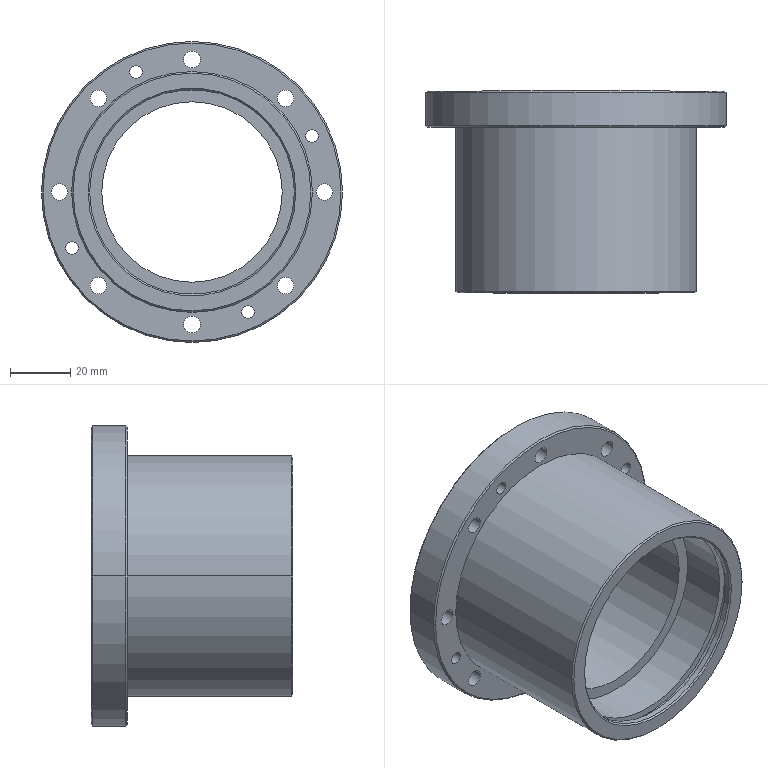Component | SolidWorks | BearingHousingAssembly-1_BearingHolder-1 | 1 solid | 85 faces | box 100 x 67 x 100 mm | volume 140911 mm3 | cylinder 58 | plane 17 | cone 10 | commonest cylinder face diameters 10 x16 5.5 x16 4.2 x8 68 x8 72.5 x4 80 x2 100 x2 60 x2 | material Plain Carbon Steel
build123d program:
from build123d import *

# Parameters (mm, degrees)
SKETCH1_R                                          = 50
BOSS_EXTRUDE1_DEPTH                                = 12
SKETCH2_R                                          = 40
BOSS_EXTRUDE2_DEPTH                                = 55
HOLE_SIZE_ACCORDING_TO_TYPE_OF_HEXAGON_D           = 5.5
HOLE_SIZE_ACCORDING_TO_TYPE_OF_HEXAGON_CBORE_D     = 10
HOLE_SIZE_ACCORDING_TO_TYPE_OF_HEXAGON_CBORE_DEPTH = 5.7
CIRPATTERN1_COUNT                                  = 8
SKETCH6_R                                          = 30
CUT_EXTRUDE1_DEPTH                                 = 98.411
SKETCH7_R                                          = 34
CUT_EXTRUDE2_DEPTH                                 = 20
CUT_EXTRUDE3_START                                 = -20
SKETCH8_R                                          = 34
CUT_EXTRUDE3_DEPTH                                 = 20
CHAMFER1_SIZE                                      = 0.5
SKETCH9_W                                          = 2.6
SKETCH9_H                                          = 2.25
M5_TAPPED_HOLE1_D                                  = 4.2
CIRPATTERN2_COUNT                                  = 4


with BuildPart() as part:
    # Sketch1 → Boss-Extrude1 (new body)
    with BuildSketch(Plane.XY):
        Circle(SKETCH1_R)
    extrude(amount=BOSS_EXTRUDE1_DEPTH)

    # Sketch2 → Boss-Extrude2 (add)
    with BuildSketch(Plane.XY.offset(12)):
        Circle(SKETCH2_R)
    extrude(amount=BOSS_EXTRUDE2_DEPTH)

    # Hole Size _according to_ type of Hexagon (through all)
    with Locations(Plane(origin=(0, 0, 0), x_dir=(-1, 0, 0), z_dir=(0, 0, -1))):
        with Locations((0, 44)):
            hole_size_according_to_type_of_hexagon = CounterBoreHole(HOLE_SIZE_ACCORDING_TO_TYPE_OF_HEXAGON_D / 2, HOLE_SIZE_ACCORDING_TO_TYPE_OF_HEXAGON_CBORE_D / 2, HOLE_SIZE_ACCORDING_TO_TYPE_OF_HEXAGON_CBORE_DEPTH)

    # CirPattern1: Hole Size _according to_ type of Hexagon ×8 about axis
    cirpattern1_axis = Axis((0, 0, 0), (0, 0, 1))
    for i in range(1, CIRPATTERN1_COUNT):
        add(hole_size_according_to_type_of_hexagon.rotate(cirpattern1_axis, i * 360 / CIRPATTERN1_COUNT), mode=Mode.SUBTRACT)

    # Sketch6 → Cut-Extrude1 (cut, through all)
    with BuildSketch(Plane.XY.offset(67)):
        Circle(SKETCH6_R)
    extrude(amount=-CUT_EXTRUDE1_DEPTH, mode=Mode.SUBTRACT)

    # Sketch7 → Cut-Extrude2 (cut)
    with BuildSketch(Plane.XY.offset(67)):
        Circle(SKETCH7_R)
    extrude(amount=-CUT_EXTRUDE2_DEPTH, mode=Mode.SUBTRACT)

    # Sketch8 → Cut-Extrude3 (cut)
    with BuildSketch(Plane(origin=(0, 0, 0), x_dir=(-1, 0, 0), z_dir=(0, 0, -1)).offset(CUT_EXTRUDE3_START)):
        with Locations(Location((0, 0, 0), (0, 0, 180))):
            Circle(SKETCH8_R)
    extrude(amount=CUT_EXTRUDE3_DEPTH, mode=Mode.SUBTRACT)

    # Chamfer1
    chamfer1_edges = [part.edges().sort_by_distance(p)[0] for p in [
        (-50, 0, 0),
        (-50, 0, 12),
        (-40, 0, 67),
        (-34, 0, 67),
        (-34, 0, 0),
    ]]
    chamfer(chamfer1_edges, length=CHAMFER1_SIZE)

    # Sketch9 → Cut-Revolve1 (revolve, cut)
    with BuildSketch(Plane(origin=(0, 0, 0), x_dir=(0, 0, -1), z_dir=(1, 0, 0)), mode=Mode.PRIVATE) as cut_revolve1_sk:
        with Locations((-63.3, 35.125)):
            Rectangle(SKETCH9_W, SKETCH9_H)
        with Locations((-3.7, 35.125)):
            Rectangle(SKETCH9_W, SKETCH9_H)
    revolve(cut_revolve1_sk.sketch.rotate(Axis((0, 0, 0), (0, 0, 1)), 90), axis=Axis((0, 0, 0), (0, 0, 1)), mode=Mode.SUBTRACT)

    # M5 Tapped Hole1 (through all)
    with Locations(Plane(origin=(0, 0, 0), x_dir=(-1, 0, 0), z_dir=(0, 0, -1))):
        with Locations((-39.878, 18.595)):
            m5_tapped_hole1 = Hole(M5_TAPPED_HOLE1_D / 2)

    # CirPattern2: M5 Tapped Hole1 ×4 about axis
    cirpattern2_axis = Axis((0, 0, 0), (0, 0, 1))
    for i in range(1, CIRPATTERN2_COUNT):
        add(m5_tapped_hole1.rotate(cirpattern2_axis, i * 360 / CIRPATTERN2_COUNT), mode=Mode.SUBTRACT)


solid = part.part

# Placed as in the assembly
solid = solid.moved(Location((-38.666, 242.264, -6), (90, 0, 0)))